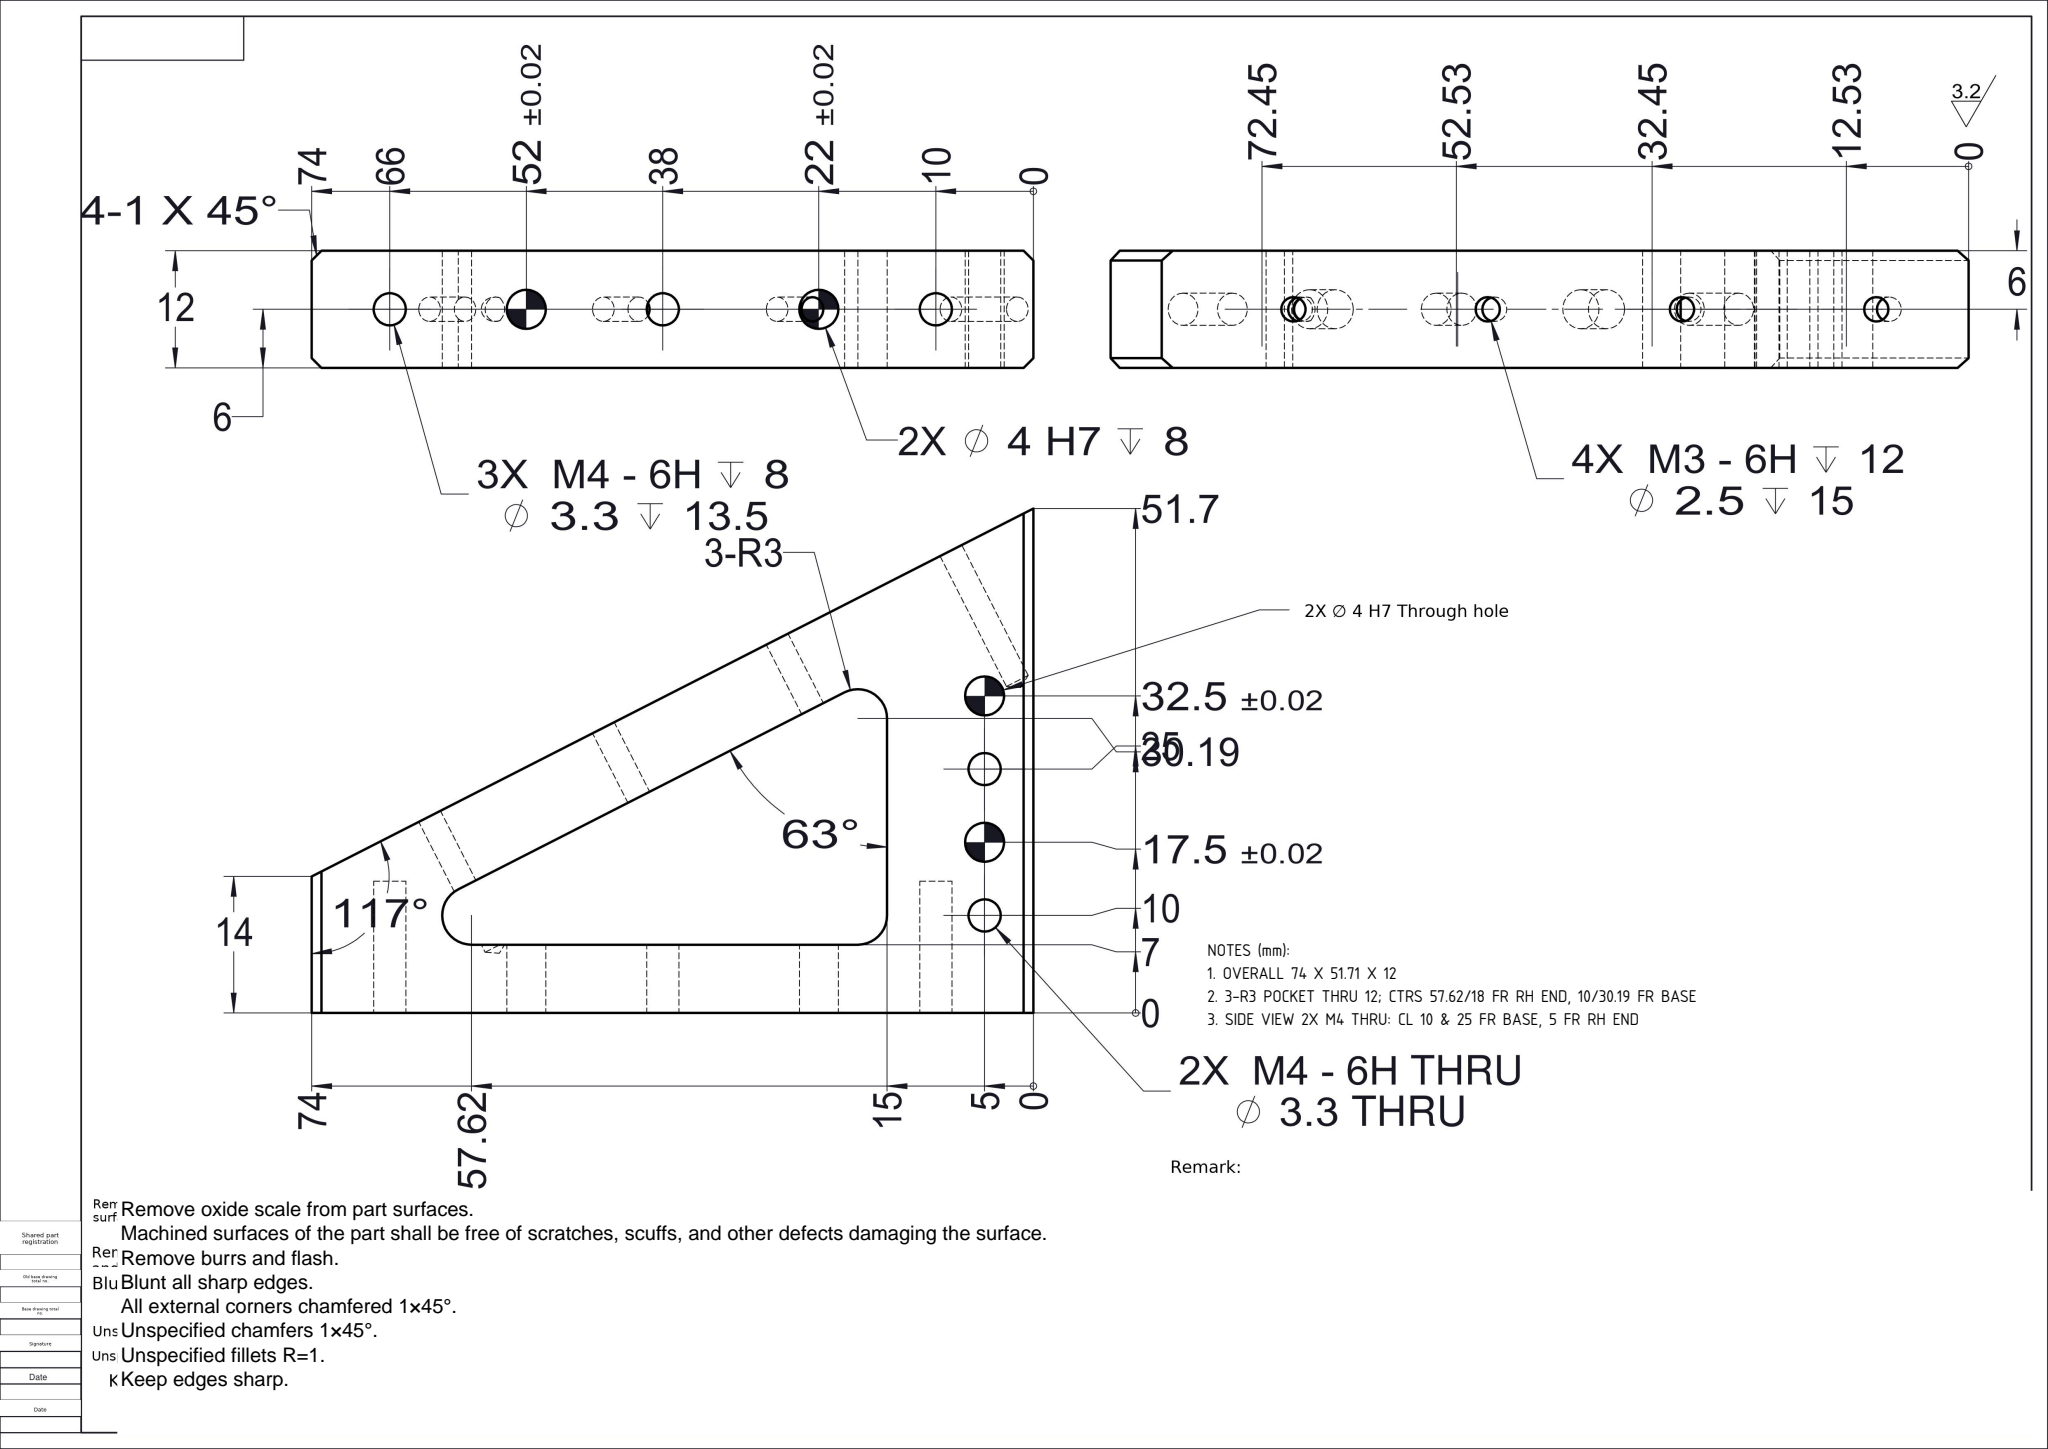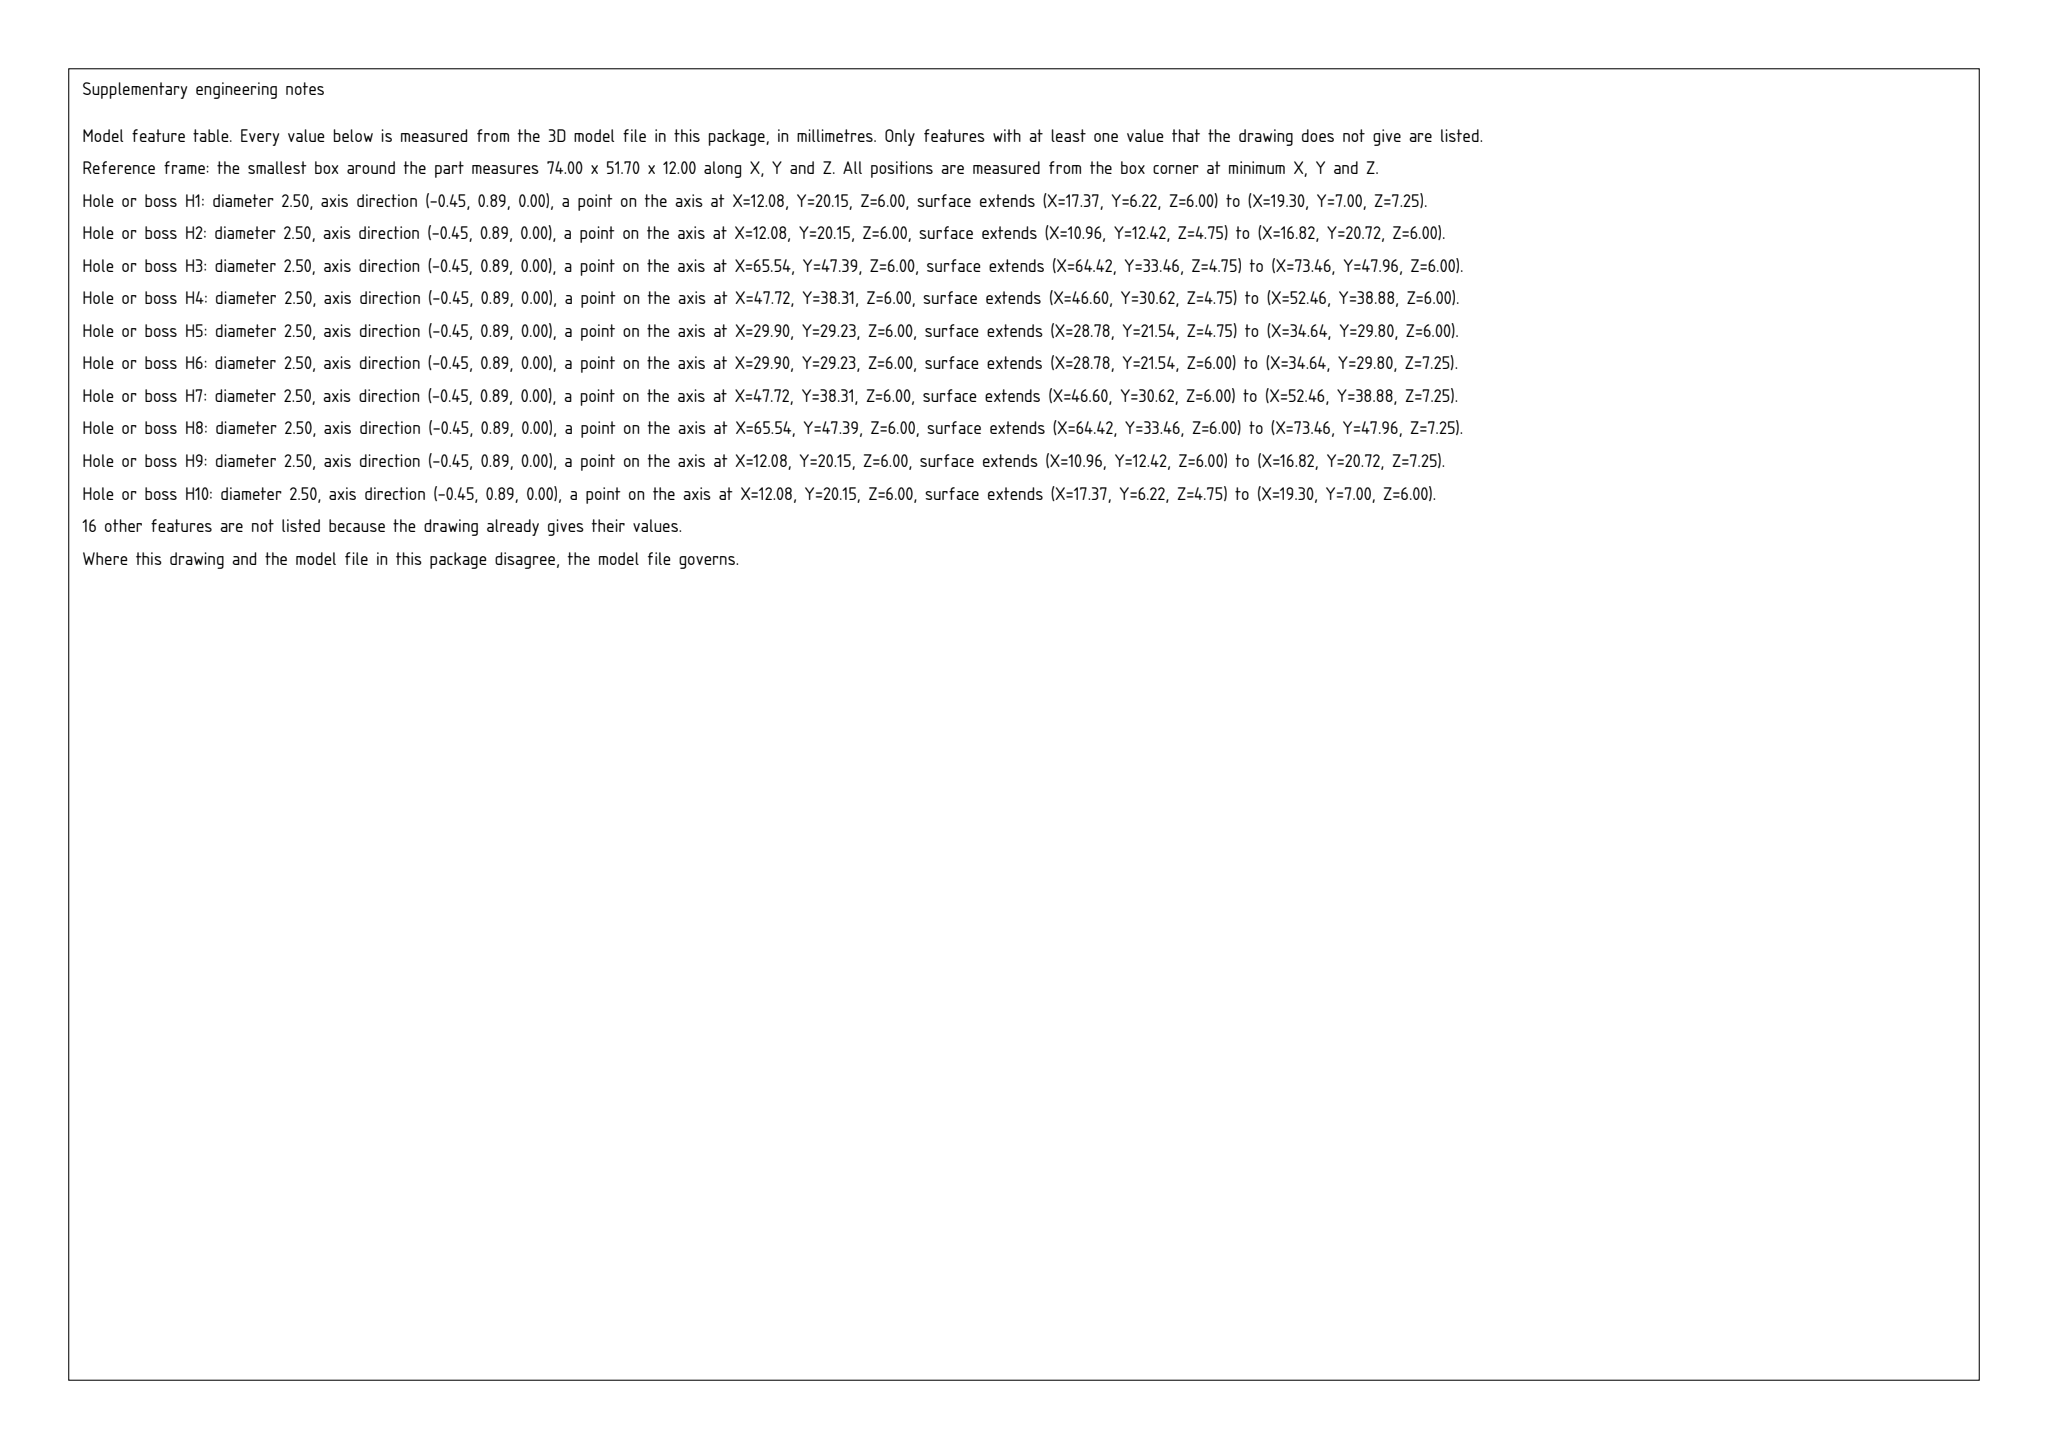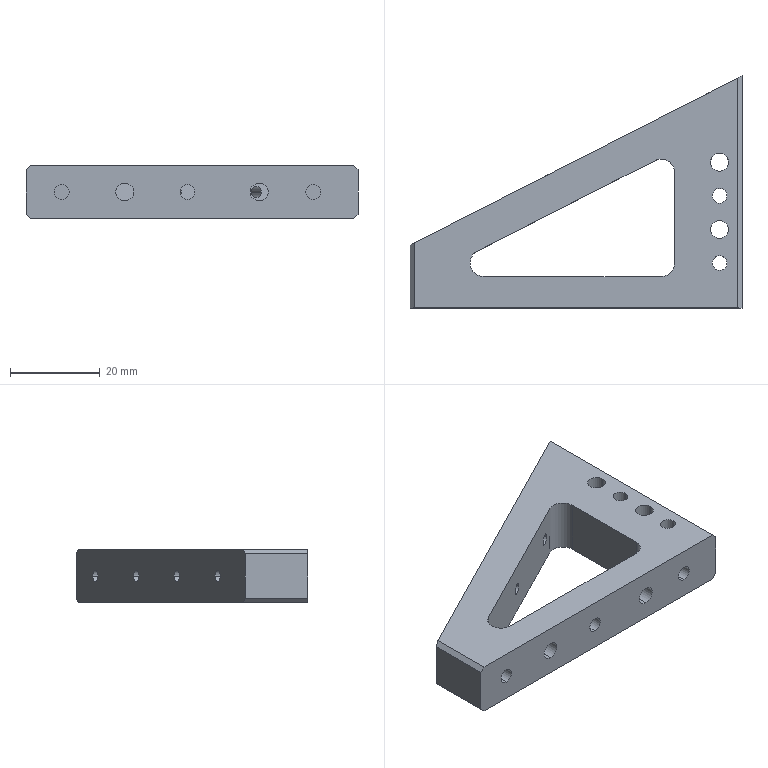Part | SolidWorks | mm | 1 solid | 51 faces | box 74 x 51.7 x 12 mm | volume 19046 mm3 | cylinder 32 | plane 15 | cone 4 | commonest cylinder face diameters 3.3 x10 2.5 x10 4 x8 6 x4
Drawing notes:
OVERALL 74 X 51.71 X 12 | from the solid: bbox_xyz [74.0, 51.705, 12.0]
3-R3 POCKET THRU 12; CTRS 57.62/18 FR RH END, 10/30.19 FR BASE | from the solid: Ø6 z-axis cyls (R3) at [16.38,10], [56,10], [56,30.19], L=12 = full thickness; 74-16.38=57.62, 74-56=18
SIDE VIEW 2X M4 THRU: CL 10 & 25 FR BASE, 5 FR RH END | from the solid: Ø3.3 z-axis cylinders at [69,10] and [69,25], L=12 thru; 74-69=5 from RH end